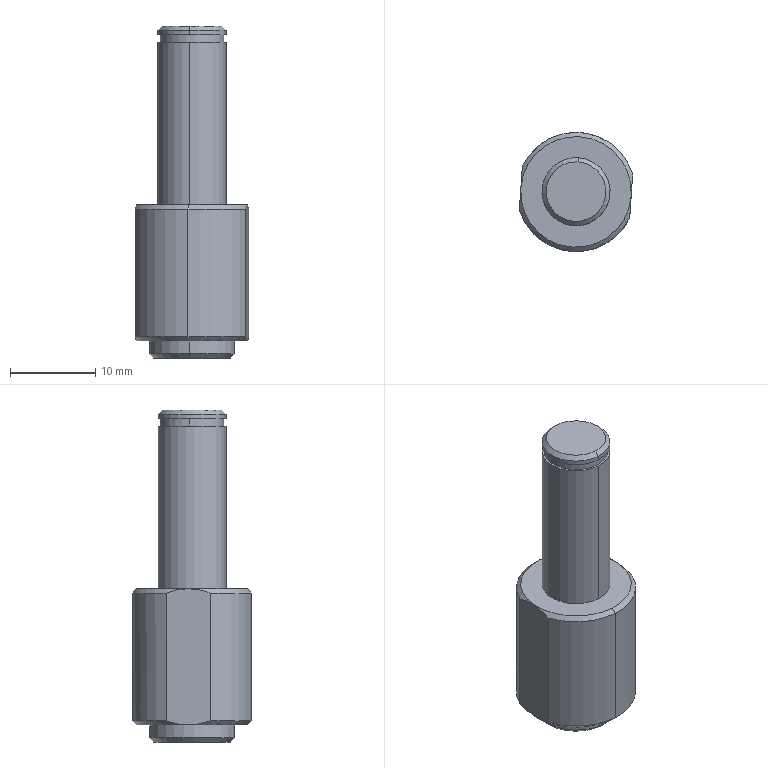Component | SolidWorks | 11-1111-1 | 1 solid | 33 faces | box 13.32 x 14 x 39 mm | volume 3399 mm3 | cylinder 13 | cone 12 | plane 8 | commonest cylinder face diameters 8 x4 14 x3 4.2 x2 7.5 x2 10 x2
STEP:
#1=CARTESIAN_POINT('',(2.505,18.513,50.79));
#2=VERTEX_POINT('',#1);
#3=CARTESIAN_POINT('',(2.529,18.867,50.79));
#4=VERTEX_POINT('',#3);
#5=CARTESIAN_POINT('',(2.517,18.69,50.79));
#6=DIRECTION('',(-0.,0.,-1.));
#7=DIRECTION('',(0.06787,0.9977,0.));
#8=AXIS2_PLACEMENT_3D('',#5,#6,#7);
#9=CIRCLE('',#8,0.1772);
#10=EDGE_CURVE('',#2,#4,#9,.T.);
#11=ORIENTED_EDGE('',*,*,#10,.F.);
#12=CARTESIAN_POINT('',(2.504,18.494,50.809));
#13=VERTEX_POINT('',#12);
#14=CARTESIAN_POINT('',(2.505,18.513,50.79));
#15=DIRECTION('',(-0.04799,-0.7055,0.7071));
#16=VECTOR('',#15,39.37);
#17=LINE('',#14,#16);
#18=EDGE_CURVE('',#2,#13,#17,.T.);
#19=ORIENTED_EDGE('',*,*,#18,.T.);
#20=CARTESIAN_POINT('',(2.53,18.886,50.809));
#21=VERTEX_POINT('',#20);
#22=CARTESIAN_POINT('',(2.517,18.69,50.809));
#23=DIRECTION('',(0.,-0.,1.));
#24=DIRECTION('',(0.06787,0.9977,0.));
#25=AXIS2_PLACEMENT_3D('',#22,#23,#24);
#26=CIRCLE('',#25,0.1969);
#27=EDGE_CURVE('',#21,#13,#26,.T.);
#28=ORIENTED_EDGE('',*,*,#27,.F.);
#29=CARTESIAN_POINT('',(2.529,18.867,50.79));
#30=DIRECTION('',(0.04799,0.7055,0.7071));
#31=VECTOR('',#30,39.37);
#32=LINE('',#29,#31);
#33=EDGE_CURVE('',#4,#21,#32,.T.);
#34=ORIENTED_EDGE('',*,*,#33,.F.);
#35=EDGE_LOOP('',(#11,#19,#28,#34));
#36=FACE_OUTER_BOUND('',#35,.T.);
#37=CARTESIAN_POINT('',(2.517,18.69,50.79));
#38=DIRECTION('',(0.,-0.,1.));
#39=DIRECTION('',(0.06787,0.9977,0.));
#40=AXIS2_PLACEMENT_3D('',#37,#38,#39);
#41=CONICAL_SURFACE('',#40,0.1772,0.7854);
#42=ADVANCED_FACE('',(#36),#41,.T.);
#43=CARTESIAN_POINT('',(2.522,18.772,51.341));
#44=VERTEX_POINT('',#43);
#45=CARTESIAN_POINT('',(2.511,18.607,51.341));
#46=VERTEX_POINT('',#45);
#47=CARTESIAN_POINT('',(2.517,18.69,51.341));
#48=DIRECTION('',(-0.,0.,-1.));
#49=DIRECTION('',(-0.06787,-0.9977,0.));
#50=AXIS2_PLACEMENT_3D('',#47,#48,#49);
#51=CIRCLE('',#50,0.08268);
#52=EDGE_CURVE('',#44,#46,#51,.T.);
#53=ORIENTED_EDGE('',*,*,#52,.F.);
#54=CARTESIAN_POINT('',(2.522,18.772,50.79));
#55=VERTEX_POINT('',#54);
#56=CARTESIAN_POINT('',(2.522,18.772,50.79));
#57=DIRECTION('',(-0.,0.,-1.));
#58=VECTOR('',#57,39.37);
#59=LINE('',#56,#58);
#60=EDGE_CURVE('',#44,#55,#59,.T.);
#61=ORIENTED_EDGE('',*,*,#60,.T.);
#62=CARTESIAN_POINT('',(2.511,18.607,50.79));
#63=VERTEX_POINT('',#62);
#64=CARTESIAN_POINT('',(2.517,18.69,50.79));
#65=DIRECTION('',(-0.,0.,-1.));
#66=DIRECTION('',(-0.06787,-0.9977,0.));
#67=AXIS2_PLACEMENT_3D('',#64,#65,#66);
#68=CIRCLE('',#67,0.08268);
#69=EDGE_CURVE('',#55,#63,#68,.T.);
#70=ORIENTED_EDGE('',*,*,#69,.T.);
#71=CARTESIAN_POINT('',(2.511,18.607,50.79));
#72=DIRECTION('',(-0.,0.,-1.));
#73=VECTOR('',#72,39.37);
#74=LINE('',#71,#73);
#75=EDGE_CURVE('',#46,#63,#74,.T.);
#76=ORIENTED_EDGE('',*,*,#75,.F.);
#77=EDGE_LOOP('',(#53,#61,#70,#76));
#78=FACE_OUTER_BOUND('',#77,.T.);
#79=CARTESIAN_POINT('',(2.517,18.69,50.79));
#80=DIRECTION('',(-0.,0.,-1.));
#81=DIRECTION('',(-0.06787,-0.9977,0.));
#82=AXIS2_PLACEMENT_3D('',#79,#80,#81);
#83=CYLINDRICAL_SURFACE('',#82,0.08268);
#84=ADVANCED_FACE('',(#78),#83,.F.);
#85=CARTESIAN_POINT('',(2.517,18.69,51.39));
#86=VERTEX_POINT('',#85);
#87=CARTESIAN_POINT('',(2.511,18.607,51.341));
#88=DIRECTION('',(-0.05818,-0.8552,-0.515));
#89=VECTOR('',#88,39.37);
#90=LINE('',#87,#89);
#91=EDGE_CURVE('',#86,#46,#90,.T.);
#92=ORIENTED_EDGE('',*,*,#91,.F.);
#93=CARTESIAN_POINT('',(2.522,18.772,51.341));
#94=DIRECTION('',(0.05818,0.8552,-0.515));
#95=VECTOR('',#94,39.37);
#96=LINE('',#93,#95);
#97=EDGE_CURVE('',#86,#44,#96,.T.);
#98=ORIENTED_EDGE('',*,*,#97,.T.);
#99=ORIENTED_EDGE('',*,*,#52,.T.);
#100=EDGE_LOOP('',(#92,#98,#99));
#101=FACE_OUTER_BOUND('',#100,.T.);
#102=CARTESIAN_POINT('',(2.517,18.69,51.341));
#103=DIRECTION('',(-0.,0.,-1.));
#104=DIRECTION('',(-0.06787,-0.9977,0.));
#105=AXIS2_PLACEMENT_3D('',#102,#103,#104);
#106=CONICAL_SURFACE('',#105,0.08268,1.03);
#107=ADVANCED_FACE('',(#101),#106,.F.);
#108=CARTESIAN_POINT('',(2.526,18.827,52.325));
#109=VERTEX_POINT('',#108);
#110=CARTESIAN_POINT('',(2.508,18.552,52.325));
#111=VERTEX_POINT('',#110);
#112=CARTESIAN_POINT('',(2.517,18.69,52.325));
#113=DIRECTION('',(0.,-0.,1.));
#114=DIRECTION('',(-0.06787,-0.9977,0.));
#115=AXIS2_PLACEMENT_3D('',#112,#113,#114);
#116=CIRCLE('',#115,0.1378);
#117=EDGE_CURVE('',#109,#111,#116,.T.);
#118=ORIENTED_EDGE('',*,*,#117,.F.);
#119=CARTESIAN_POINT('',(2.528,18.847,52.305));
#120=VERTEX_POINT('',#119);
#121=CARTESIAN_POINT('',(2.528,18.847,52.305));
#122=DIRECTION('',(0.04799,0.7055,-0.7071));
#123=VECTOR('',#122,39.37);
#124=LINE('',#121,#123);
#125=EDGE_CURVE('',#109,#120,#124,.T.);
#126=ORIENTED_EDGE('',*,*,#125,.T.);
#127=CARTESIAN_POINT('',(2.506,18.533,52.305));
#128=VERTEX_POINT('',#127);
#129=CARTESIAN_POINT('',(2.517,18.69,52.305));
#130=DIRECTION('',(-0.,0.,-1.));
#131=DIRECTION('',(-0.06787,-0.9977,0.));
#132=AXIS2_PLACEMENT_3D('',#129,#130,#131);
#133=CIRCLE('',#132,0.1575);
#134=EDGE_CURVE('',#128,#120,#133,.T.);
#135=ORIENTED_EDGE('',*,*,#134,.F.);
#136=CARTESIAN_POINT('',(2.506,18.533,52.305));
#137=DIRECTION('',(-0.04799,-0.7055,-0.7071));
#138=VECTOR('',#137,39.37);
#139=LINE('',#136,#138);
#140=EDGE_CURVE('',#111,#128,#139,.T.);
#141=ORIENTED_EDGE('',*,*,#140,.F.);
#142=EDGE_LOOP('',(#118,#126,#135,#141));
#143=FACE_OUTER_BOUND('',#142,.T.);
#144=CARTESIAN_POINT('',(2.517,18.69,52.305));
#145=DIRECTION('',(-0.,0.,-1.));
#146=DIRECTION('',(-0.06787,-0.9977,0.));
#147=AXIS2_PLACEMENT_3D('',#144,#145,#146);
#148=CONICAL_SURFACE('',#147,0.1575,0.7854);
#149=ADVANCED_FACE('',(#143),#148,.T.);
#150=ORIENTED_EDGE('',*,*,#134,.T.);
#151=CARTESIAN_POINT('',(2.528,18.847,52.286));
#152=VERTEX_POINT('',#151);
#153=CARTESIAN_POINT('',(2.528,18.847,50.79));
#154=DIRECTION('',(-0.,0.,-1.));
#155=VECTOR('',#154,39.37);
#156=LINE('',#153,#155);
#157=EDGE_CURVE('',#120,#152,#156,.T.);
#158=ORIENTED_EDGE('',*,*,#157,.T.);
#159=CARTESIAN_POINT('',(2.506,18.533,52.286));
#160=VERTEX_POINT('',#159);
#161=CARTESIAN_POINT('',(2.517,18.69,52.286));
#162=DIRECTION('',(0.,-0.,1.));
#163=DIRECTION('',(-0.9977,0.06787,0.));
#164=AXIS2_PLACEMENT_3D('',#161,#162,#163);
#165=CIRCLE('',#164,0.1575);
#166=EDGE_CURVE('',#152,#160,#165,.T.);
#167=ORIENTED_EDGE('',*,*,#166,.T.);
#168=CARTESIAN_POINT('',(2.506,18.533,50.79));
#169=DIRECTION('',(-0.,0.,-1.));
#170=VECTOR('',#169,39.37);
#171=LINE('',#168,#170);
#172=EDGE_CURVE('',#128,#160,#171,.T.);
#173=ORIENTED_EDGE('',*,*,#172,.F.);
#174=EDGE_LOOP('',(#150,#158,#167,#173));
#175=FACE_OUTER_BOUND('',#174,.T.);
#176=CARTESIAN_POINT('',(2.517,18.69,50.79));
#177=DIRECTION('',(-0.,0.,-1.));
#178=DIRECTION('',(-0.06787,-0.9977,0.));
#179=AXIS2_PLACEMENT_3D('',#176,#177,#178);
#180=CYLINDRICAL_SURFACE('',#179,0.1575);
#181=ADVANCED_FACE('',(#175),#180,.T.);
#182=CARTESIAN_POINT('',(2.37,18.7,52.25));
#183=VERTEX_POINT('',#182);
#184=CARTESIAN_POINT('',(2.664,18.68,52.25));
#185=VERTEX_POINT('',#184);
#186=CARTESIAN_POINT('',(2.517,18.69,52.25));
#187=DIRECTION('',(0.,-0.,1.));
#188=DIRECTION('',(-0.9977,0.06787,0.));
#189=AXIS2_PLACEMENT_3D('',#186,#187,#188);
#190=CIRCLE('',#189,0.1476);
#191=EDGE_CURVE('',#183,#185,#190,.T.);
#192=ORIENTED_EDGE('',*,*,#191,.T.);
#193=CARTESIAN_POINT('',(2.664,18.68,52.286));
#194=VERTEX_POINT('',#193);
#195=CARTESIAN_POINT('',(2.664,18.68,52.25));
#196=DIRECTION('',(0.,-0.,1.));
#197=VECTOR('',#196,39.37);
#198=LINE('',#195,#197);
#199=EDGE_CURVE('',#185,#194,#198,.T.);
#200=ORIENTED_EDGE('',*,*,#199,.T.);
#201=CARTESIAN_POINT('',(2.37,18.7,52.286));
#202=VERTEX_POINT('',#201);
#203=CARTESIAN_POINT('',(2.517,18.69,52.286));
#204=DIRECTION('',(0.,-0.,1.));
#205=DIRECTION('',(-0.9977,0.06787,0.));
#206=AXIS2_PLACEMENT_3D('',#203,#204,#205);
#207=CIRCLE('',#206,0.1476);
#208=EDGE_CURVE('',#202,#194,#207,.T.);
#209=ORIENTED_EDGE('',*,*,#208,.F.);
#210=CARTESIAN_POINT('',(2.37,18.7,52.25));
#211=DIRECTION('',(0.,-0.,1.));
#212=VECTOR('',#211,39.37);
#213=LINE('',#210,#212);
#214=EDGE_CURVE('',#183,#202,#213,.T.);
#215=ORIENTED_EDGE('',*,*,#214,.F.);
#216=EDGE_LOOP('',(#192,#200,#209,#215));
#217=FACE_OUTER_BOUND('',#216,.T.);
#218=CARTESIAN_POINT('',(2.517,18.69,52.25));
#219=DIRECTION('',(0.,-0.,1.));
#220=DIRECTION('',(-0.9977,0.06787,0.));
#221=AXIS2_PLACEMENT_3D('',#218,#219,#220);
#222=CYLINDRICAL_SURFACE('',#221,0.1476);
#223=ADVANCED_FACE('',(#217),#222,.T.);
#224=CARTESIAN_POINT('',(2.504,18.494,50.868));
#225=VERTEX_POINT('',#224);
#226=CARTESIAN_POINT('',(2.53,18.886,50.868));
#227=VERTEX_POINT('',#226);
#228=CARTESIAN_POINT('',(2.517,18.69,50.868));
#229=DIRECTION('',(-0.,0.,-1.));
#230=DIRECTION('',(-0.06787,-0.9977,0.));
#231=AXIS2_PLACEMENT_3D('',#228,#229,#230);
#232=CIRCLE('',#231,0.1969);
#233=EDGE_CURVE('',#225,#227,#232,.T.);
#234=ORIENTED_EDGE('',*,*,#233,.T.);
#235=CARTESIAN_POINT('',(2.53,18.886,50.79));
#236=DIRECTION('',(-0.,0.,-1.));
#237=VECTOR('',#236,39.37);
#238=LINE('',#235,#237);
#239=EDGE_CURVE('',#227,#21,#238,.T.);
#240=ORIENTED_EDGE('',*,*,#239,.T.);
#241=ORIENTED_EDGE('',*,*,#27,.T.);
#242=CARTESIAN_POINT('',(2.504,18.494,50.79));
#243=DIRECTION('',(-0.,0.,-1.));
#244=VECTOR('',#243,39.37);
#245=LINE('',#242,#244);
#246=EDGE_CURVE('',#225,#13,#245,.T.);
#247=ORIENTED_EDGE('',*,*,#246,.F.);
#248=EDGE_LOOP('',(#234,#240,#241,#247));
#249=FACE_OUTER_BOUND('',#248,.T.);
#250=CARTESIAN_POINT('',(2.517,18.69,50.79));
#251=DIRECTION('',(-0.,0.,-1.));
#252=DIRECTION('',(-0.06787,-0.9977,0.));
#253=AXIS2_PLACEMENT_3D('',#250,#251,#252);
#254=CYLINDRICAL_SURFACE('',#253,0.1969);
#255=ADVANCED_FACE('',(#249),#254,.T.);
#256=CARTESIAN_POINT('',(2.528,18.847,52.25));
#257=VERTEX_POINT('',#256);
#258=CARTESIAN_POINT('',(2.506,18.533,52.25));
#259=VERTEX_POINT('',#258);
#260=CARTESIAN_POINT('',(2.517,18.69,52.25));
#261=DIRECTION('',(0.,-0.,1.));
#262=DIRECTION('',(-0.9977,0.06787,0.));
#263=AXIS2_PLACEMENT_3D('',#260,#261,#262);
#264=CIRCLE('',#263,0.1575);
#265=EDGE_CURVE('',#257,#259,#264,.T.);
#266=ORIENTED_EDGE('',*,*,#265,.F.);
#267=CARTESIAN_POINT('',(2.528,18.847,51.498));
#268=VERTEX_POINT('',#267);
#269=CARTESIAN_POINT('',(2.528,18.847,50.79));
#270=DIRECTION('',(-0.,0.,-1.));
#271=VECTOR('',#270,39.37);
#272=LINE('',#269,#271);
#273=EDGE_CURVE('',#257,#268,#272,.T.);
#274=ORIENTED_EDGE('',*,*,#273,.T.);
#275=CARTESIAN_POINT('',(2.506,18.533,51.498));
#276=VERTEX_POINT('',#275);
#277=CARTESIAN_POINT('',(2.517,18.69,51.498));
#278=DIRECTION('',(-0.,0.,-1.));
#279=DIRECTION('',(-0.06787,-0.9977,0.));
#280=AXIS2_PLACEMENT_3D('',#277,#278,#279);
#281=CIRCLE('',#280,0.1575);
#282=EDGE_CURVE('',#276,#268,#281,.T.);
#283=ORIENTED_EDGE('',*,*,#282,.F.);
#284=CARTESIAN_POINT('',(2.506,18.533,50.79));
#285=DIRECTION('',(-0.,0.,-1.));
#286=VECTOR('',#285,39.37);
#287=LINE('',#284,#286);
#288=EDGE_CURVE('',#259,#276,#287,.T.);
#289=ORIENTED_EDGE('',*,*,#288,.F.);
#290=EDGE_LOOP('',(#266,#274,#283,#289));
#291=FACE_OUTER_BOUND('',#290,.T.);
#292=CARTESIAN_POINT('',(2.517,18.69,50.79));
#293=DIRECTION('',(-0.,0.,-1.));
#294=DIRECTION('',(-0.06787,-0.9977,0.));
#295=AXIS2_PLACEMENT_3D('',#292,#293,#294);
#296=CYLINDRICAL_SURFACE('',#295,0.1575);
#297=ADVANCED_FACE('',(#291),#296,.T.);
#298=CARTESIAN_POINT('',(2.499,18.435,51.498));
#299=VERTEX_POINT('',#298);
#300=CARTESIAN_POINT('',(2.772,18.673,51.498));
#301=VERTEX_POINT('',#300);
#302=CARTESIAN_POINT('',(2.517,18.69,51.498));
#303=DIRECTION('',(0.,-0.,1.));
#304=DIRECTION('',(-0.06787,-0.9977,0.));
#305=AXIS2_PLACEMENT_3D('',#302,#303,#304);
#306=CIRCLE('',#305,0.2559);
#307=EDGE_CURVE('',#299,#301,#306,.T.);
#308=ORIENTED_EDGE('',*,*,#307,.F.);
#309=CARTESIAN_POINT('',(2.498,18.415,51.479));
#310=VERTEX_POINT('',#309);
#311=CARTESIAN_POINT('',(2.498,18.415,51.479));
#312=DIRECTION('',(-0.04799,-0.7055,-0.7071));
#313=VECTOR('',#312,39.37);
#314=LINE('',#311,#313);
#315=EDGE_CURVE('',#299,#310,#314,.T.);
#316=ORIENTED_EDGE('',*,*,#315,.T.);
#317=CARTESIAN_POINT('',(2.765,18.571,51.479));
#318=VERTEX_POINT('',#317);
#319=CARTESIAN_POINT('',(2.517,18.69,51.479));
#320=DIRECTION('',(-0.,0.,-1.));
#321=DIRECTION('',(-0.06787,-0.9977,0.));
#322=AXIS2_PLACEMENT_3D('',#319,#320,#321);
#323=CIRCLE('',#322,0.2756);
#324=EDGE_CURVE('',#318,#310,#323,.T.);
#325=ORIENTED_EDGE('',*,*,#324,.F.);
#326=CARTESIAN_POINT('',(2.765,18.571,51.479));
#327=CARTESIAN_POINT('',(2.766,18.587,51.485));
#328=CARTESIAN_POINT('',(2.767,18.604,51.49));
#329=CARTESIAN_POINT('',(2.769,18.629,51.495));
#330=CARTESIAN_POINT('',(2.77,18.638,51.496));
#331=CARTESIAN_POINT('',(2.771,18.655,51.498));
#332=CARTESIAN_POINT('',(2.772,18.664,51.498));
#333=CARTESIAN_POINT('',(2.772,18.673,51.498));
#334=B_SPLINE_CURVE_WITH_KNOTS('',3,(#326,#327,#328,#329,#330,#331,#332,#333),.UNSPECIFIED.,.F.,.F.,(4,2,2,4),(0.005495,0.00681,0.007467,0.008124),.UNSPECIFIED.);
#335=EDGE_CURVE('',#318,#301,#334,.T.);
#336=ORIENTED_EDGE('',*,*,#335,.T.);
#337=EDGE_LOOP('',(#308,#316,#325,#336));
#338=FACE_OUTER_BOUND('',#337,.T.);
#339=CARTESIAN_POINT('',(2.517,18.69,51.479));
#340=DIRECTION('',(-0.,0.,-1.));
#341=DIRECTION('',(-0.06787,-0.9977,0.));
#342=AXIS2_PLACEMENT_3D('',#339,#340,#341);
#343=CONICAL_SURFACE('',#342,0.2756,0.7854);
#344=ADVANCED_FACE('',(#338),#343,.T.);
#345=CARTESIAN_POINT('',(2.534,18.945,50.868));
#346=VERTEX_POINT('',#345);
#347=CARTESIAN_POINT('',(2.772,18.673,50.868));
#348=VERTEX_POINT('',#347);
#349=CARTESIAN_POINT('',(2.517,18.69,50.868));
#350=DIRECTION('',(-0.,0.,-1.));
#351=DIRECTION('',(0.06787,0.9977,0.));
#352=AXIS2_PLACEMENT_3D('',#349,#350,#351);
#353=CIRCLE('',#352,0.2559);
#354=EDGE_CURVE('',#346,#348,#353,.T.);
#355=ORIENTED_EDGE('',*,*,#354,.F.);
#356=CARTESIAN_POINT('',(2.536,18.965,50.888));
#357=VERTEX_POINT('',#356);
#358=CARTESIAN_POINT('',(2.534,18.945,50.868));
#359=DIRECTION('',(0.04799,0.7055,0.7071));
#360=VECTOR('',#359,39.37);
#361=LINE('',#358,#360);
#362=EDGE_CURVE('',#346,#357,#361,.T.);
#363=ORIENTED_EDGE('',*,*,#362,.T.);
#364=CARTESIAN_POINT('',(2.779,18.775,50.888));
#365=VERTEX_POINT('',#364);
#366=CARTESIAN_POINT('',(2.517,18.69,50.888));
#367=DIRECTION('',(0.,-0.,1.));
#368=DIRECTION('',(0.06787,0.9977,0.));
#369=AXIS2_PLACEMENT_3D('',#366,#367,#368);
#370=CIRCLE('',#369,0.2756);
#371=EDGE_CURVE('',#365,#357,#370,.T.);
#372=ORIENTED_EDGE('',*,*,#371,.F.);
#373=CARTESIAN_POINT('',(2.779,18.775,50.888));
#374=CARTESIAN_POINT('',(2.779,18.766,50.885));
#375=CARTESIAN_POINT('',(2.778,18.758,50.882));
#376=CARTESIAN_POINT('',(2.777,18.741,50.877));
#377=CARTESIAN_POINT('',(2.776,18.733,50.875));
#378=CARTESIAN_POINT('',(2.775,18.707,50.87));
#379=CARTESIAN_POINT('',(2.773,18.69,50.868));
#380=CARTESIAN_POINT('',(2.772,18.673,50.868));
#381=B_SPLINE_CURVE_WITH_KNOTS('',3,(#373,#374,#375,#376,#377,#378,#379,#380),.UNSPECIFIED.,.F.,.F.,(4,2,2,4),(0.0025,0.003161,0.003821,0.005143),.UNSPECIFIED.);
#382=EDGE_CURVE('',#365,#348,#381,.T.);
#383=ORIENTED_EDGE('',*,*,#382,.T.);
#384=EDGE_LOOP('',(#355,#363,#372,#383));
#385=FACE_OUTER_BOUND('',#384,.T.);
#386=CARTESIAN_POINT('',(2.517,18.69,50.868));
#387=DIRECTION('',(0.,-0.,1.));
#388=DIRECTION('',(0.06787,0.9977,0.));
#389=AXIS2_PLACEMENT_3D('',#386,#387,#388);
#390=CONICAL_SURFACE('',#389,0.2559,0.7854);
#391=ADVANCED_FACE('',(#385),#390,.T.);
#392=ORIENTED_EDGE('',*,*,#324,.T.);
#393=CARTESIAN_POINT('',(2.498,18.415,50.888));
#394=VERTEX_POINT('',#393);
#395=CARTESIAN_POINT('',(2.498,18.415,50.79));
#396=DIRECTION('',(-0.,0.,-1.));
#397=VECTOR('',#396,39.37);
#398=LINE('',#395,#397);
#399=EDGE_CURVE('',#310,#394,#398,.T.);
#400=ORIENTED_EDGE('',*,*,#399,.T.);
#401=CARTESIAN_POINT('',(2.765,18.571,50.888));
#402=VERTEX_POINT('',#401);
#403=CARTESIAN_POINT('',(2.517,18.69,50.888));
#404=DIRECTION('',(0.,-0.,1.));
#405=DIRECTION('',(0.06787,0.9977,0.));
#406=AXIS2_PLACEMENT_3D('',#403,#404,#405);
#407=CIRCLE('',#406,0.2756);
#408=EDGE_CURVE('',#394,#402,#407,.T.);
#409=ORIENTED_EDGE('',*,*,#408,.T.);
#410=CARTESIAN_POINT('',(2.765,18.571,50.79));
#411=DIRECTION('',(-0.,0.,-1.));
#412=VECTOR('',#411,39.37);
#413=LINE('',#410,#412);
#414=EDGE_CURVE('',#318,#402,#413,.T.);
#415=ORIENTED_EDGE('',*,*,#414,.F.);
#416=EDGE_LOOP('',(#392,#400,#409,#415));
#417=FACE_OUTER_BOUND('',#416,.T.);
#418=CARTESIAN_POINT('',(2.517,18.69,50.79));
#419=DIRECTION('',(-0.,0.,-1.));
#420=DIRECTION('',(-0.06787,-0.9977,0.));
#421=AXIS2_PLACEMENT_3D('',#418,#419,#420);
#422=CYLINDRICAL_SURFACE('',#421,0.2756);
#423=ADVANCED_FACE('',(#417),#422,.T.);
#424=CARTESIAN_POINT('',(2.268,18.809,51.479));
#425=VERTEX_POINT('',#424);
#426=CARTESIAN_POINT('',(2.268,18.809,50.888));
#427=VERTEX_POINT('',#426);
#428=CARTESIAN_POINT('',(2.268,18.809,50.79));
#429=DIRECTION('',(-0.,0.,-1.));
#430=VECTOR('',#429,39.37);
#431=LINE('',#428,#430);
#432=EDGE_CURVE('',#425,#427,#431,.T.);
#433=ORIENTED_EDGE('',*,*,#432,.F.);
#434=CARTESIAN_POINT('',(2.779,18.775,51.479));
#435=VERTEX_POINT('',#434);
#436=CARTESIAN_POINT('',(2.517,18.69,51.479));
#437=DIRECTION('',(-0.,0.,-1.));
#438=DIRECTION('',(-0.06787,-0.9977,0.));
#439=AXIS2_PLACEMENT_3D('',#436,#437,#438);
#440=CIRCLE('',#439,0.2756);
#441=EDGE_CURVE('',#425,#435,#440,.T.);
#442=ORIENTED_EDGE('',*,*,#441,.T.);
#443=CARTESIAN_POINT('',(2.779,18.775,50.79));
#444=DIRECTION('',(0.,-0.,1.));
#445=VECTOR('',#444,39.37);
#446=LINE('',#443,#445);
#447=EDGE_CURVE('',#365,#435,#446,.T.);
#448=ORIENTED_EDGE('',*,*,#447,.F.);
#449=ORIENTED_EDGE('',*,*,#371,.T.);
#450=CARTESIAN_POINT('',(2.517,18.69,50.888));
#451=DIRECTION('',(0.,-0.,1.));
#452=DIRECTION('',(0.06787,0.9977,0.));
#453=AXIS2_PLACEMENT_3D('',#450,#451,#452);
#454=CIRCLE('',#453,0.2756);
#455=EDGE_CURVE('',#357,#427,#454,.T.);
#456=ORIENTED_EDGE('',*,*,#455,.T.);
#457=EDGE_LOOP('',(#433,#442,#448,#449,#456));
#458=FACE_OUTER_BOUND('',#457,.T.);
#459=CARTESIAN_POINT('',(2.517,18.69,50.79));
#460=DIRECTION('',(-0.,0.,-1.));
#461=DIRECTION('',(-0.06787,-0.9977,0.));
#462=AXIS2_PLACEMENT_3D('',#459,#460,#461);
#463=CYLINDRICAL_SURFACE('',#462,0.2756);
#464=ADVANCED_FACE('',(#458),#463,.T.);
#465=ORIENTED_EDGE('',*,*,#399,.F.);
#466=CARTESIAN_POINT('',(2.255,18.605,51.479));
#467=VERTEX_POINT('',#466);
#468=CARTESIAN_POINT('',(2.517,18.69,51.479));
#469=DIRECTION('',(-0.,0.,-1.));
#470=DIRECTION('',(-0.06787,-0.9977,0.));
#471=AXIS2_PLACEMENT_3D('',#468,#469,#470);
#472=CIRCLE('',#471,0.2756);
#473=EDGE_CURVE('',#310,#467,#472,.T.);
#474=ORIENTED_EDGE('',*,*,#473,.T.);
#475=CARTESIAN_POINT('',(2.255,18.605,50.888));
#476=VERTEX_POINT('',#475);
#477=CARTESIAN_POINT('',(2.255,18.605,50.79));
#478=DIRECTION('',(0.,-0.,1.));
#479=VECTOR('',#478,39.37);
#480=LINE('',#477,#479);
#481=EDGE_CURVE('',#476,#467,#480,.T.);
#482=ORIENTED_EDGE('',*,*,#481,.F.);
#483=CARTESIAN_POINT('',(2.517,18.69,50.888));
#484=DIRECTION('',(0.,-0.,1.));
#485=DIRECTION('',(0.06787,0.9977,0.));
#486=AXIS2_PLACEMENT_3D('',#483,#484,#485);
#487=CIRCLE('',#486,0.2756);
#488=EDGE_CURVE('',#476,#394,#487,.T.);
#489=ORIENTED_EDGE('',*,*,#488,.T.);
#490=EDGE_LOOP('',(#465,#474,#482,#489));
#491=FACE_OUTER_BOUND('',#490,.T.);
#492=CARTESIAN_POINT('',(2.517,18.69,50.79));
#493=DIRECTION('',(-0.,0.,-1.));
#494=DIRECTION('',(-0.06787,-0.9977,0.));
#495=AXIS2_PLACEMENT_3D('',#492,#493,#494);
#496=CYLINDRICAL_SURFACE('',#495,0.2756);
#497=ADVANCED_FACE('',(#491),#496,.T.);
#498=ORIENTED_EDGE('',*,*,#488,.F.);
#499=CARTESIAN_POINT('',(2.262,18.707,50.868));
#500=VERTEX_POINT('',#499);
#501=CARTESIAN_POINT('',(2.255,18.605,50.888));
#502=CARTESIAN_POINT('',(2.256,18.622,50.882));
#503=CARTESIAN_POINT('',(2.257,18.638,50.877));
#504=CARTESIAN_POINT('',(2.259,18.664,50.872));
#505=CARTESIAN_POINT('',(2.259,18.672,50.871));
#506=CARTESIAN_POINT('',(2.26,18.69,50.869));
#507=CARTESIAN_POINT('',(2.261,18.699,50.868));
#508=CARTESIAN_POINT('',(2.262,18.707,50.868));
#509=B_SPLINE_CURVE_WITH_KNOTS('',3,(#501,#502,#503,#504,#505,#506,#507,#508),.UNSPECIFIED.,.F.,.F.,(4,2,2,4),(0.005495,0.00681,0.007467,0.008124),.UNSPECIFIED.);
#510=EDGE_CURVE('',#476,#500,#509,.T.);
#511=ORIENTED_EDGE('',*,*,#510,.T.);
#512=CARTESIAN_POINT('',(2.517,18.69,50.868));
#513=DIRECTION('',(-0.,0.,-1.));
#514=DIRECTION('',(0.06787,0.9977,0.));
#515=AXIS2_PLACEMENT_3D('',#512,#513,#514);
#516=CIRCLE('',#515,0.2559);
#517=EDGE_CURVE('',#348,#500,#516,.T.);
#518=ORIENTED_EDGE('',*,*,#517,.F.);
#519=CARTESIAN_POINT('',(2.772,18.673,50.868));
#520=CARTESIAN_POINT('',(2.772,18.664,50.868));
#521=CARTESIAN_POINT('',(2.771,18.655,50.869));
#522=CARTESIAN_POINT('',(2.77,18.638,50.871));
#523=CARTESIAN_POINT('',(2.769,18.629,50.872));
#524=CARTESIAN_POINT('',(2.767,18.604,50.877));
#525=CARTESIAN_POINT('',(2.766,18.587,50.882));
#526=CARTESIAN_POINT('',(2.765,18.571,50.888));
#527=B_SPLINE_CURVE_WITH_KNOTS('',3,(#519,#520,#521,#522,#523,#524,#525,#526),.UNSPECIFIED.,.F.,.F.,(4,2,2,4),(0.005143,0.005804,0.006465,0.007787),.UNSPECIFIED.);
#528=EDGE_CURVE('',#348,#402,#527,.T.);
#529=ORIENTED_EDGE('',*,*,#528,.T.);
#530=ORIENTED_EDGE('',*,*,#408,.F.);
#531=EDGE_LOOP('',(#498,#511,#518,#529,#530));
#532=FACE_OUTER_BOUND('',#531,.T.);
#533=CARTESIAN_POINT('',(2.517,18.69,50.868));
#534=DIRECTION('',(0.,-0.,1.));
#535=DIRECTION('',(0.06787,0.9977,0.));
#536=AXIS2_PLACEMENT_3D('',#533,#534,#535);
#537=CONICAL_SURFACE('',#536,0.2559,0.7854);
#538=ADVANCED_FACE('',(#532),#537,.T.);
#539=ORIENTED_EDGE('',*,*,#362,.F.);
#540=CARTESIAN_POINT('',(2.517,18.69,50.868));
#541=DIRECTION('',(-0.,0.,-1.));
#542=DIRECTION('',(0.06787,0.9977,0.));
#543=AXIS2_PLACEMENT_3D('',#540,#541,#542);
#544=CIRCLE('',#543,0.2559);
#545=EDGE_CURVE('',#500,#346,#544,.T.);
#546=ORIENTED_EDGE('',*,*,#545,.F.);
#547=CARTESIAN_POINT('',(2.262,18.707,50.868));
#548=CARTESIAN_POINT('',(2.263,18.725,50.868));
#549=CARTESIAN_POINT('',(2.264,18.742,50.87));
#550=CARTESIAN_POINT('',(2.266,18.768,50.875));
#551=CARTESIAN_POINT('',(2.266,18.776,50.877));
#552=CARTESIAN_POINT('',(2.267,18.793,50.882));
#553=CARTESIAN_POINT('',(2.268,18.801,50.885));
#554=CARTESIAN_POINT('',(2.268,18.809,50.888));
#555=B_SPLINE_CURVE_WITH_KNOTS('',3,(#547,#548,#549,#550,#551,#552,#553,#554),.UNSPECIFIED.,.F.,.F.,(4,2,2,4),(0.008124,0.009438,0.01009,0.01075),.UNSPECIFIED.);
#556=EDGE_CURVE('',#500,#427,#555,.T.);
#557=ORIENTED_EDGE('',*,*,#556,.T.);
#558=ORIENTED_EDGE('',*,*,#455,.F.);
#559=EDGE_LOOP('',(#539,#546,#557,#558));
#560=FACE_OUTER_BOUND('',#559,.T.);
#561=CARTESIAN_POINT('',(2.517,18.69,50.868));
#562=DIRECTION('',(0.,-0.,1.));
#563=DIRECTION('',(0.06787,0.9977,0.));
#564=AXIS2_PLACEMENT_3D('',#561,#562,#563);
#565=CONICAL_SURFACE('',#564,0.2559,0.7854);
#566=ADVANCED_FACE('',(#560),#565,.T.);
#567=ORIENTED_EDGE('',*,*,#441,.F.);
#568=CARTESIAN_POINT('',(2.262,18.707,51.498));
#569=VERTEX_POINT('',#568);
#570=CARTESIAN_POINT('',(2.268,18.809,51.479));
#571=CARTESIAN_POINT('',(2.268,18.801,51.482));
#572=CARTESIAN_POINT('',(2.267,18.793,51.484));
#573=CARTESIAN_POINT('',(2.266,18.776,51.489));
#574=CARTESIAN_POINT('',(2.266,18.768,51.491));
#575=CARTESIAN_POINT('',(2.264,18.742,51.496));
#576=CARTESIAN_POINT('',(2.263,18.725,51.498));
#577=CARTESIAN_POINT('',(2.262,18.707,51.498));
#578=B_SPLINE_CURVE_WITH_KNOTS('',3,(#570,#571,#572,#573,#574,#575,#576,#577),.UNSPECIFIED.,.F.,.F.,(4,2,2,4),(0.0025,0.003161,0.003821,0.005143),.UNSPECIFIED.);
#579=EDGE_CURVE('',#425,#569,#578,.T.);
#580=ORIENTED_EDGE('',*,*,#579,.T.);
#581=CARTESIAN_POINT('',(2.517,18.69,51.498));
#582=DIRECTION('',(0.,-0.,1.));
#583=DIRECTION('',(-0.06787,-0.9977,0.));
#584=AXIS2_PLACEMENT_3D('',#581,#582,#583);
#585=CIRCLE('',#584,0.2559);
#586=EDGE_CURVE('',#301,#569,#585,.T.);
#587=ORIENTED_EDGE('',*,*,#586,.F.);
#588=CARTESIAN_POINT('',(2.772,18.673,51.498));
#589=CARTESIAN_POINT('',(2.773,18.69,51.498));
#590=CARTESIAN_POINT('',(2.775,18.707,51.496));
#591=CARTESIAN_POINT('',(2.776,18.733,51.491));
#592=CARTESIAN_POINT('',(2.777,18.741,51.489));
#593=CARTESIAN_POINT('',(2.778,18.758,51.484));
#594=CARTESIAN_POINT('',(2.779,18.766,51.482));
#595=CARTESIAN_POINT('',(2.779,18.775,51.479));
#596=B_SPLINE_CURVE_WITH_KNOTS('',3,(#588,#589,#590,#591,#592,#593,#594,#595),.UNSPECIFIED.,.F.,.F.,(4,2,2,4),(0.008124,0.009438,0.01009,0.01075),.UNSPECIFIED.);
#597=EDGE_CURVE('',#301,#435,#596,.T.);
#598=ORIENTED_EDGE('',*,*,#597,.T.);
#599=EDGE_LOOP('',(#567,#580,#587,#598));
#600=FACE_OUTER_BOUND('',#599,.T.);
#601=CARTESIAN_POINT('',(2.517,18.69,51.479));
#602=DIRECTION('',(-0.,0.,-1.));
#603=DIRECTION('',(-0.06787,-0.9977,0.));
#604=AXIS2_PLACEMENT_3D('',#601,#602,#603);
#605=CONICAL_SURFACE('',#604,0.2756,0.7854);
#606=ADVANCED_FACE('',(#600),#605,.T.);
#607=ORIENTED_EDGE('',*,*,#315,.F.);
#608=CARTESIAN_POINT('',(2.517,18.69,51.498));
#609=DIRECTION('',(0.,-0.,1.));
#610=DIRECTION('',(-0.06787,-0.9977,0.));
#611=AXIS2_PLACEMENT_3D('',#608,#609,#610);
#612=CIRCLE('',#611,0.2559);
#613=EDGE_CURVE('',#569,#299,#612,.T.);
#614=ORIENTED_EDGE('',*,*,#613,.F.);
#615=CARTESIAN_POINT('',(2.262,18.707,51.498));
#616=CARTESIAN_POINT('',(2.261,18.699,51.498));
#617=CARTESIAN_POINT('',(2.26,18.69,51.498));
#618=CARTESIAN_POINT('',(2.259,18.672,51.496));
#619=CARTESIAN_POINT('',(2.259,18.664,51.495));
#620=CARTESIAN_POINT('',(2.257,18.638,51.49));
#621=CARTESIAN_POINT('',(2.256,18.622,51.485));
#622=CARTESIAN_POINT('',(2.255,18.605,51.479));
#623=B_SPLINE_CURVE_WITH_KNOTS('',3,(#615,#616,#617,#618,#619,#620,#621,#622),.UNSPECIFIED.,.F.,.F.,(4,2,2,4),(0.005143,0.005804,0.006465,0.007787),.UNSPECIFIED.);
#624=EDGE_CURVE('',#569,#467,#623,.T.);
#625=ORIENTED_EDGE('',*,*,#624,.T.);
#626=ORIENTED_EDGE('',*,*,#473,.F.);
#627=EDGE_LOOP('',(#607,#614,#625,#626));
#628=FACE_OUTER_BOUND('',#627,.T.);
#629=CARTESIAN_POINT('',(2.517,18.69,51.479));
#630=DIRECTION('',(-0.,0.,-1.));
#631=DIRECTION('',(-0.06787,-0.9977,0.));
#632=AXIS2_PLACEMENT_3D('',#629,#630,#631);
#633=CONICAL_SURFACE('',#632,0.2756,0.7854);
#634=ADVANCED_FACE('',(#628),#633,.T.);
#635=ORIENTED_EDGE('',*,*,#273,.F.);
#636=CARTESIAN_POINT('',(2.517,18.69,52.25));
#637=DIRECTION('',(0.,-0.,1.));
#638=DIRECTION('',(-0.9977,0.06787,0.));
#639=AXIS2_PLACEMENT_3D('',#636,#637,#638);
#640=CIRCLE('',#639,0.1575);
#641=EDGE_CURVE('',#259,#257,#640,.T.);
#642=ORIENTED_EDGE('',*,*,#641,.F.);
#643=ORIENTED_EDGE('',*,*,#288,.T.);
#644=CARTESIAN_POINT('',(2.517,18.69,51.498));
#645=DIRECTION('',(-0.,0.,-1.));
#646=DIRECTION('',(-0.06787,-0.9977,0.));
#647=AXIS2_PLACEMENT_3D('',#644,#645,#646);
#648=CIRCLE('',#647,0.1575);
#649=EDGE_CURVE('',#268,#276,#648,.T.);
#650=ORIENTED_EDGE('',*,*,#649,.F.);
#651=EDGE_LOOP('',(#635,#642,#643,#650));
#652=FACE_OUTER_BOUND('',#651,.T.);
#653=CARTESIAN_POINT('',(2.517,18.69,50.79));
#654=DIRECTION('',(-0.,0.,-1.));
#655=DIRECTION('',(-0.06787,-0.9977,0.));
#656=AXIS2_PLACEMENT_3D('',#653,#654,#655);
#657=CYLINDRICAL_SURFACE('',#656,0.1575);
#658=ADVANCED_FACE('',(#652),#657,.T.);
#659=ORIENTED_EDGE('',*,*,#586,.T.);
#660=ORIENTED_EDGE('',*,*,#613,.T.);
#661=ORIENTED_EDGE('',*,*,#307,.T.);
#662=EDGE_LOOP('',(#659,#660,#661));
#663=FACE_OUTER_BOUND('',#662,.T.);
#664=ORIENTED_EDGE('',*,*,#282,.T.);
#665=ORIENTED_EDGE('',*,*,#649,.T.);
#666=EDGE_LOOP('',(#664,#665));
#667=FACE_BOUND('',#666,.T.);
#668=CARTESIAN_POINT('',(2.528,18.847,51.498));
#669=DIRECTION('',(-0.,0.,-1.));
#670=DIRECTION('',(-0.06787,-0.9977,-0.));
#671=AXIS2_PLACEMENT_3D('',#668,#669,#670);
#672=PLANE('',#671);
#673=ADVANCED_FACE('',(#663,#667),#672,.F.);
#674=ORIENTED_EDGE('',*,*,#517,.T.);
#675=ORIENTED_EDGE('',*,*,#545,.T.);
#676=ORIENTED_EDGE('',*,*,#354,.T.);
#677=EDGE_LOOP('',(#674,#675,#676));
#678=FACE_OUTER_BOUND('',#677,.T.);
#679=ORIENTED_EDGE('',*,*,#233,.F.);
#680=CARTESIAN_POINT('',(2.517,18.69,50.868));
#681=DIRECTION('',(-0.,0.,-1.));
#682=DIRECTION('',(-0.06787,-0.9977,0.));
#683=AXIS2_PLACEMENT_3D('',#680,#681,#682);
#684=CIRCLE('',#683,0.1969);
#685=EDGE_CURVE('',#227,#225,#684,.T.);
#686=ORIENTED_EDGE('',*,*,#685,.F.);
#687=EDGE_LOOP('',(#679,#686));
#688=FACE_BOUND('',#687,.T.);
#689=CARTESIAN_POINT('',(2.536,18.965,50.868));
#690=DIRECTION('',(0.,-0.,1.));
#691=DIRECTION('',(0.06787,0.9977,0.));
#692=AXIS2_PLACEMENT_3D('',#689,#690,#691);
#693=PLANE('',#692);
#694=ADVANCED_FACE('',(#678,#688),#693,.F.);
#695=ORIENTED_EDGE('',*,*,#239,.F.);
#696=ORIENTED_EDGE('',*,*,#685,.T.);
#697=ORIENTED_EDGE('',*,*,#246,.T.);
#698=CARTESIAN_POINT('',(2.517,18.69,50.809));
#699=DIRECTION('',(0.,-0.,1.));
#700=DIRECTION('',(0.06787,0.9977,0.));
#701=AXIS2_PLACEMENT_3D('',#698,#699,#700);
#702=CIRCLE('',#701,0.1969);
#703=EDGE_CURVE('',#13,#21,#702,.T.);
#704=ORIENTED_EDGE('',*,*,#703,.T.);
#705=EDGE_LOOP('',(#695,#696,#697,#704));
#706=FACE_OUTER_BOUND('',#705,.T.);
#707=CARTESIAN_POINT('',(2.517,18.69,50.79));
#708=DIRECTION('',(-0.,0.,-1.));
#709=DIRECTION('',(-0.06787,-0.9977,0.));
#710=AXIS2_PLACEMENT_3D('',#707,#708,#709);
#711=CYLINDRICAL_SURFACE('',#710,0.1969);
#712=ADVANCED_FACE('',(#706),#711,.T.);
#713=CARTESIAN_POINT('',(2.517,18.69,50.79));
#714=DIRECTION('',(-0.,0.,-1.));
#715=DIRECTION('',(0.06787,0.9977,0.));
#716=AXIS2_PLACEMENT_3D('',#713,#714,#715);
#717=CIRCLE('',#716,0.1772);
#718=EDGE_CURVE('',#4,#2,#717,.T.);
#719=ORIENTED_EDGE('',*,*,#718,.T.);
#720=ORIENTED_EDGE('',*,*,#10,.T.);
#721=EDGE_LOOP('',(#719,#720));
#722=FACE_OUTER_BOUND('',#721,.T.);
#723=CARTESIAN_POINT('',(2.517,18.69,50.79));
#724=DIRECTION('',(-0.,0.,-1.));
#725=DIRECTION('',(-0.06787,-0.9977,0.));
#726=AXIS2_PLACEMENT_3D('',#723,#724,#725);
#727=CIRCLE('',#726,0.08268);
#728=EDGE_CURVE('',#63,#55,#727,.T.);
#729=ORIENTED_EDGE('',*,*,#728,.F.);
#730=ORIENTED_EDGE('',*,*,#69,.F.);
#731=EDGE_LOOP('',(#729,#730));
#732=FACE_BOUND('',#731,.T.);
#733=CARTESIAN_POINT('',(2.53,18.886,50.79));
#734=DIRECTION('',(0.,-0.,1.));
#735=DIRECTION('',(0.06787,0.9977,0.));
#736=AXIS2_PLACEMENT_3D('',#733,#734,#735);
#737=PLANE('',#736);
#738=ADVANCED_FACE('',(#722,#732),#737,.F.);
#739=ORIENTED_EDGE('',*,*,#191,.F.);
#740=CARTESIAN_POINT('',(2.517,18.69,52.25));
#741=DIRECTION('',(0.,-0.,1.));
#742=DIRECTION('',(-0.9977,0.06787,0.));
#743=AXIS2_PLACEMENT_3D('',#740,#741,#742);
#744=CIRCLE('',#743,0.1476);
#745=EDGE_CURVE('',#185,#183,#744,.T.);
#746=ORIENTED_EDGE('',*,*,#745,.F.);
#747=EDGE_LOOP('',(#739,#746));
#748=FACE_BOUND('',#747,.T.);
#749=ORIENTED_EDGE('',*,*,#641,.T.);
#750=ORIENTED_EDGE('',*,*,#265,.T.);
#751=EDGE_LOOP('',(#749,#750));
#752=FACE_OUTER_BOUND('',#751,.T.);
#753=CARTESIAN_POINT('',(2.517,18.69,52.25));
#754=DIRECTION('',(0.,-0.,1.));
#755=DIRECTION('',(-0.9977,0.06787,0.));
#756=AXIS2_PLACEMENT_3D('',#753,#754,#755);
#757=PLANE('',#756);
#758=ADVANCED_FACE('',(#748,#752),#757,.T.);
#759=ORIENTED_EDGE('',*,*,#208,.T.);
#760=CARTESIAN_POINT('',(2.517,18.69,52.286));
#761=DIRECTION('',(0.,-0.,1.));
#762=DIRECTION('',(-0.9977,0.06787,0.));
#763=AXIS2_PLACEMENT_3D('',#760,#761,#762);
#764=CIRCLE('',#763,0.1476);
#765=EDGE_CURVE('',#194,#202,#764,.T.);
#766=ORIENTED_EDGE('',*,*,#765,.T.);
#767=EDGE_LOOP('',(#759,#766));
#768=FACE_BOUND('',#767,.T.);
#769=CARTESIAN_POINT('',(2.517,18.69,52.286));
#770=DIRECTION('',(0.,-0.,1.));
#771=DIRECTION('',(-0.9977,0.06787,0.));
#772=AXIS2_PLACEMENT_3D('',#769,#770,#771);
#773=CIRCLE('',#772,0.1575);
#774=EDGE_CURVE('',#160,#152,#773,.T.);
#775=ORIENTED_EDGE('',*,*,#774,.F.);
#776=ORIENTED_EDGE('',*,*,#166,.F.);
#777=EDGE_LOOP('',(#775,#776));
#778=FACE_OUTER_BOUND('',#777,.T.);
#779=CARTESIAN_POINT('',(2.517,18.69,52.286));
#780=DIRECTION('',(0.,-0.,1.));
#781=DIRECTION('',(-0.9977,0.06787,0.));
#782=AXIS2_PLACEMENT_3D('',#779,#780,#781);
#783=PLANE('',#782);
#784=ADVANCED_FACE('',(#768,#778),#783,.F.);
#785=ORIENTED_EDGE('',*,*,#199,.F.);
#786=ORIENTED_EDGE('',*,*,#745,.T.);
#787=ORIENTED_EDGE('',*,*,#214,.T.);
#788=ORIENTED_EDGE('',*,*,#765,.F.);
#789=EDGE_LOOP('',(#785,#786,#787,#788));
#790=FACE_OUTER_BOUND('',#789,.T.);
#791=CARTESIAN_POINT('',(2.517,18.69,52.25));
#792=DIRECTION('',(0.,-0.,1.));
#793=DIRECTION('',(-0.9977,0.06787,0.));
#794=AXIS2_PLACEMENT_3D('',#791,#792,#793);
#795=CYLINDRICAL_SURFACE('',#794,0.1476);
#796=ADVANCED_FACE('',(#790),#795,.T.);
#797=CARTESIAN_POINT('',(2.517,18.69,52.325));
#798=DIRECTION('',(0.,-0.,1.));
#799=DIRECTION('',(-0.06787,-0.9977,0.));
#800=AXIS2_PLACEMENT_3D('',#797,#798,#799);
#801=CIRCLE('',#800,0.1378);
#802=EDGE_CURVE('',#111,#109,#801,.T.);
#803=ORIENTED_EDGE('',*,*,#802,.T.);
#804=ORIENTED_EDGE('',*,*,#117,.T.);
#805=EDGE_LOOP('',(#803,#804));
#806=FACE_OUTER_BOUND('',#805,.T.);
#807=CARTESIAN_POINT('',(2.517,18.69,52.325));
#808=DIRECTION('',(-0.,0.,-1.));
#809=DIRECTION('',(-0.06787,-0.9977,-0.));
#810=AXIS2_PLACEMENT_3D('',#807,#808,#809);
#811=PLANE('',#810);
#812=ADVANCED_FACE('',(#806),#811,.F.);
#813=ORIENTED_EDGE('',*,*,#157,.F.);
#814=CARTESIAN_POINT('',(2.517,18.69,52.305));
#815=DIRECTION('',(-0.,0.,-1.));
#816=DIRECTION('',(-0.06787,-0.9977,0.));
#817=AXIS2_PLACEMENT_3D('',#814,#815,#816);
#818=CIRCLE('',#817,0.1575);
#819=EDGE_CURVE('',#120,#128,#818,.T.);
#820=ORIENTED_EDGE('',*,*,#819,.T.);
#821=ORIENTED_EDGE('',*,*,#172,.T.);
#822=ORIENTED_EDGE('',*,*,#774,.T.);
#823=EDGE_LOOP('',(#813,#820,#821,#822));
#824=FACE_OUTER_BOUND('',#823,.T.);
#825=CARTESIAN_POINT('',(2.517,18.69,50.79));
#826=DIRECTION('',(-0.,0.,-1.));
#827=DIRECTION('',(-0.06787,-0.9977,0.));
#828=AXIS2_PLACEMENT_3D('',#825,#826,#827);
#829=CYLINDRICAL_SURFACE('',#828,0.1575);
#830=ADVANCED_FACE('',(#824),#829,.T.);
#831=ORIENTED_EDGE('',*,*,#125,.F.);
#832=ORIENTED_EDGE('',*,*,#802,.F.);
#833=ORIENTED_EDGE('',*,*,#140,.T.);
#834=ORIENTED_EDGE('',*,*,#819,.F.);
#835=EDGE_LOOP('',(#831,#832,#833,#834));
#836=FACE_OUTER_BOUND('',#835,.T.);
#837=CARTESIAN_POINT('',(2.517,18.69,52.305));
#838=DIRECTION('',(-0.,0.,-1.));
#839=DIRECTION('',(-0.06787,-0.9977,0.));
#840=AXIS2_PLACEMENT_3D('',#837,#838,#839);
#841=CONICAL_SURFACE('',#840,0.1575,0.7854);
#842=ADVANCED_FACE('',(#836),#841,.T.);
#843=ORIENTED_EDGE('',*,*,#97,.F.);
#844=ORIENTED_EDGE('',*,*,#91,.T.);
#845=CARTESIAN_POINT('',(2.517,18.69,51.341));
#846=DIRECTION('',(-0.,0.,-1.));
#847=DIRECTION('',(-0.06787,-0.9977,0.));
#848=AXIS2_PLACEMENT_3D('',#845,#846,#847);
#849=CIRCLE('',#848,0.08268);
#850=EDGE_CURVE('',#46,#44,#849,.T.);
#851=ORIENTED_EDGE('',*,*,#850,.T.);
#852=EDGE_LOOP('',(#843,#844,#851));
#853=FACE_OUTER_BOUND('',#852,.T.);
#854=CARTESIAN_POINT('',(2.517,18.69,51.341));
#855=DIRECTION('',(-0.,0.,-1.));
#856=DIRECTION('',(-0.06787,-0.9977,0.));
#857=AXIS2_PLACEMENT_3D('',#854,#855,#856);
#858=CONICAL_SURFACE('',#857,0.08268,1.03);
#859=ADVANCED_FACE('',(#853),#858,.F.);
#860=ORIENTED_EDGE('',*,*,#60,.F.);
#861=ORIENTED_EDGE('',*,*,#850,.F.);
#862=ORIENTED_EDGE('',*,*,#75,.T.);
#863=ORIENTED_EDGE('',*,*,#728,.T.);
#864=EDGE_LOOP('',(#860,#861,#862,#863));
#865=FACE_OUTER_BOUND('',#864,.T.);
#866=CARTESIAN_POINT('',(2.517,18.69,50.79));
#867=DIRECTION('',(-0.,0.,-1.));
#868=DIRECTION('',(-0.06787,-0.9977,0.));
#869=AXIS2_PLACEMENT_3D('',#866,#867,#868);
#870=CYLINDRICAL_SURFACE('',#869,0.08268);
#871=ADVANCED_FACE('',(#865),#870,.F.);
#872=ORIENTED_EDGE('',*,*,#447,.T.);
#873=ORIENTED_EDGE('',*,*,#597,.F.);
#874=ORIENTED_EDGE('',*,*,#335,.F.);
#875=ORIENTED_EDGE('',*,*,#414,.T.);
#876=ORIENTED_EDGE('',*,*,#528,.F.);
#877=ORIENTED_EDGE('',*,*,#382,.F.);
#878=EDGE_LOOP('',(#872,#873,#874,#875,#876,#877));
#879=FACE_OUTER_BOUND('',#878,.T.);
#880=CARTESIAN_POINT('',(2.812,19.262,52.325));
#881=DIRECTION('',(0.9977,-0.06787,-0.));
#882=DIRECTION('',(0.,-0.,1.));
#883=AXIS2_PLACEMENT_3D('',#880,#881,#882);
#884=PLANE('',#883);
#885=ADVANCED_FACE('',(#879),#884,.T.);
#886=ORIENTED_EDGE('',*,*,#481,.T.);
#887=ORIENTED_EDGE('',*,*,#624,.F.);
#888=ORIENTED_EDGE('',*,*,#579,.F.);
#889=ORIENTED_EDGE('',*,*,#432,.T.);
#890=ORIENTED_EDGE('',*,*,#556,.F.);
#891=ORIENTED_EDGE('',*,*,#510,.F.);
#892=EDGE_LOOP('',(#886,#887,#888,#889,#890,#891));
#893=FACE_OUTER_BOUND('',#892,.T.);
#894=CARTESIAN_POINT('',(2.302,19.296,52.325));
#895=DIRECTION('',(-0.9977,0.06787,0.));
#896=DIRECTION('',(-0.,0.,-1.));
#897=AXIS2_PLACEMENT_3D('',#894,#895,#896);
#898=PLANE('',#897);
#899=ADVANCED_FACE('',(#893),#898,.T.);
#900=ORIENTED_EDGE('',*,*,#18,.F.);
#901=ORIENTED_EDGE('',*,*,#718,.F.);
#902=ORIENTED_EDGE('',*,*,#33,.T.);
#903=ORIENTED_EDGE('',*,*,#703,.F.);
#904=EDGE_LOOP('',(#900,#901,#902,#903));
#905=FACE_OUTER_BOUND('',#904,.T.);
#906=CARTESIAN_POINT('',(2.517,18.69,50.79));
#907=DIRECTION('',(0.,-0.,1.));
#908=DIRECTION('',(0.06787,0.9977,0.));
#909=AXIS2_PLACEMENT_3D('',#906,#907,#908);
#910=CONICAL_SURFACE('',#909,0.1772,0.7854);
#911=ADVANCED_FACE('',(#905),#910,.T.);
#912=CLOSED_SHELL('',(#42,#84,#107,#149,#181,#223,#255,#297,#344,#391,#423,#464,#497,#538,#566,#606,#634,#658,#673,#694,#712,#738,#758,#784,#796,#812,#830,#842,#859,#871,#885,#899,#911));
#913=MANIFOLD_SOLID_BREP('',#912);
#914=CARTESIAN_POINT('',(0.,0.,0.));
#915=DIRECTION('',(0.,0.,1.));
#916=DIRECTION('',(1.,0.,0.));
#917=AXIS2_PLACEMENT_3D('',#914,#915,#916);
#918=(LENGTH_UNIT()NAMED_UNIT(*)SI_UNIT($,.METRE.));
#919=LENGTH_MEASURE_WITH_UNIT(LENGTH_MEASURE(0.0254),#918);
#920=DIMENSIONAL_EXPONENTS(1.,0.,0.,0.,0.,0.,0.);
#921=(CONVERSION_BASED_UNIT('',#919)LENGTH_UNIT()NAMED_UNIT(#920));
#922=UNCERTAINTY_MEASURE_WITH_UNIT(LENGTH_MEASURE(0.00001),#921,'','');
#923=(NAMED_UNIT(*)PLANE_ANGLE_UNIT()SI_UNIT($,.RADIAN.));
#924=(NAMED_UNIT(*)SI_UNIT($,.STERADIAN.)SOLID_ANGLE_UNIT());
#925=(GEOMETRIC_REPRESENTATION_CONTEXT(3)GLOBAL_UNCERTAINTY_ASSIGNED_CONTEXT((#922))GLOBAL_UNIT_ASSIGNED_CONTEXT((#921,#923,#924))REPRESENTATION_CONTEXT('',''));
#926=ADVANCED_BREP_SHAPE_REPRESENTATION('',(#913,#917),#925);
#927=COLOUR_RGB('',0.7922,0.8196,0.9333);
#928=FILL_AREA_STYLE_COLOUR('',#927);
#929=FILL_AREA_STYLE('',(#928));
#930=SURFACE_STYLE_FILL_AREA(#929);
#931=SURFACE_SIDE_STYLE('',(#930));
#932=SURFACE_STYLE_USAGE(.BOTH.,#931);
#933=PRESENTATION_STYLE_ASSIGNMENT((#932));
#934=STYLED_ITEM('',(#933),#913);
#935=(LENGTH_UNIT()NAMED_UNIT(*)SI_UNIT($,.METRE.));
#936=LENGTH_MEASURE_WITH_UNIT(LENGTH_MEASURE(0.0254),#935);
#937=DIMENSIONAL_EXPONENTS(1.,0.,0.,0.,0.,0.,0.);
#938=(CONVERSION_BASED_UNIT('',#936)LENGTH_UNIT()NAMED_UNIT(#937));
#939=UNCERTAINTY_MEASURE_WITH_UNIT(LENGTH_MEASURE(0.00001),#938,'','');
#940=(NAMED_UNIT(*)PLANE_ANGLE_UNIT()SI_UNIT($,.RADIAN.));
#941=(NAMED_UNIT(*)SI_UNIT($,.STERADIAN.)SOLID_ANGLE_UNIT());
#942=(GEOMETRIC_REPRESENTATION_CONTEXT(3)GLOBAL_UNCERTAINTY_ASSIGNED_CONTEXT((#939))GLOBAL_UNIT_ASSIGNED_CONTEXT((#938,#940,#941))REPRESENTATION_CONTEXT('',''));
#943=MECHANICAL_DESIGN_GEOMETRIC_PRESENTATION_REPRESENTATION('',(#934),#942);
#944=PRESENTATION_LAYER_ASSIGNMENT('','',(#934));